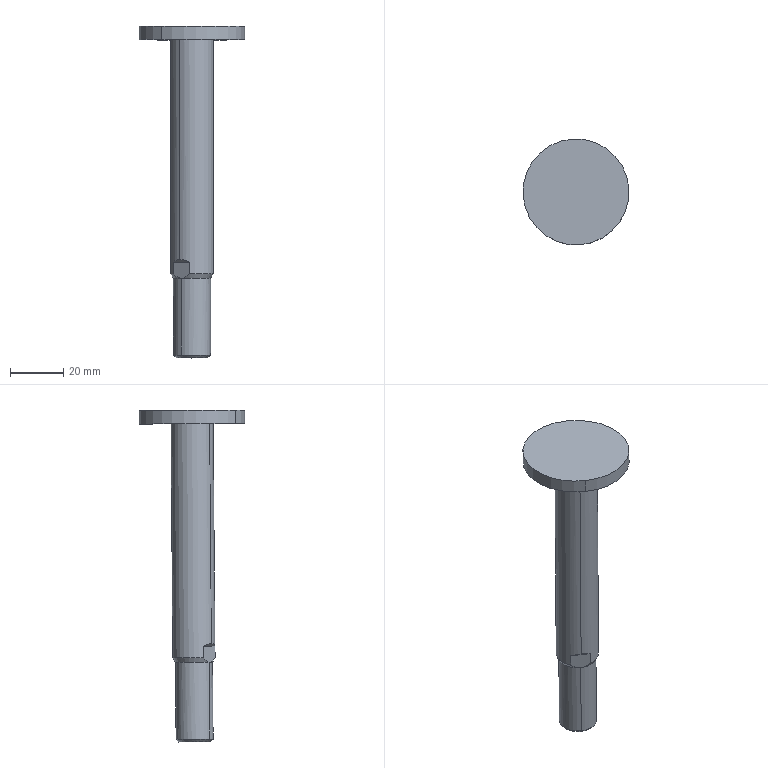Component | SolidWorks | CG1UN40-50Piston-1 | 1 solid | 17 faces | box 40 x 40.04 x 125.21 mm | volume 28878 mm3 | plane 7 | cylinder 6 | cone 4 | commonest cylinder face diameters 16 x2 40 x2 14 x2
STEP:
#1=CARTESIAN_POINT('',(8.156,4.289,0.9635));
#2=VERTEX_POINT('',#1);
#3=CARTESIAN_POINT('',(8.053,4.409,1.002));
#4=VERTEX_POINT('',#3);
#5=CARTESIAN_POINT('',(8.156,4.289,0.9635));
#6=CARTESIAN_POINT('',(8.132,4.338,0.9891));
#7=CARTESIAN_POINT('',(8.097,4.378,1.002));
#8=CARTESIAN_POINT('',(8.053,4.409,1.002));
#9=(BOUNDED_CURVE()B_SPLINE_CURVE(3,(#5,#6,#7,#8),.UNSPECIFIED.,.F.,.F.)B_SPLINE_CURVE_WITH_KNOTS((4,4),(5.778,6.283),.UNSPECIFIED.)CURVE()GEOMETRIC_REPRESENTATION_ITEM()RATIONAL_B_SPLINE_CURVE((1.,0.9788,0.9788,1.))REPRESENTATION_ITEM(''));
#10=EDGE_CURVE('',#2,#4,#9,.T.);
#11=ORIENTED_EDGE('',*,*,#10,.T.);
#12=CARTESIAN_POINT('',(8.053,4.435,4.27));
#13=VERTEX_POINT('',#12);
#14=CARTESIAN_POINT('',(8.053,4.42,2.439));
#15=DIRECTION('',(-0.,0.008055,1.));
#16=VECTOR('',#15,39.37);
#17=LINE('',#14,#16);
#18=EDGE_CURVE('',#4,#13,#17,.T.);
#19=ORIENTED_EDGE('',*,*,#18,.T.);
#20=CARTESIAN_POINT('',(7.695,3.917,4.274));
#21=VERTEX_POINT('',#20);
#22=CARTESIAN_POINT('',(7.874,4.176,4.272));
#23=DIRECTION('',(0.,-0.008055,-1.));
#24=DIRECTION('',(-0.5679,-0.823,0.00663));
#25=AXIS2_PLACEMENT_3D('',#22,#23,#24);
#26=CIRCLE('',#25,0.315);
#27=EDGE_CURVE('',#13,#21,#26,.T.);
#28=ORIENTED_EDGE('',*,*,#27,.T.);
#29=CARTESIAN_POINT('',(7.695,3.89,1.006));
#30=VERTEX_POINT('',#29);
#31=CARTESIAN_POINT('',(7.695,3.902,2.443));
#32=DIRECTION('',(-0.,0.008055,1.));
#33=VECTOR('',#32,39.37);
#34=LINE('',#31,#33);
#35=EDGE_CURVE('',#30,#21,#34,.T.);
#36=ORIENTED_EDGE('',*,*,#35,.F.);
#37=CARTESIAN_POINT('',(7.843,3.836,0.9672));
#38=VERTEX_POINT('',#37);
#39=CARTESIAN_POINT('',(7.695,3.89,1.006));
#40=CARTESIAN_POINT('',(7.739,3.86,1.006));
#41=CARTESIAN_POINT('',(7.79,3.841,0.9931));
#42=CARTESIAN_POINT('',(7.843,3.836,0.9672));
#43=(BOUNDED_CURVE()B_SPLINE_CURVE(3,(#39,#40,#41,#42),.UNSPECIFIED.,.F.,.T.)B_SPLINE_CURVE_WITH_KNOTS((4,4),(0.,0.5054),.UNSPECIFIED.)CURVE()GEOMETRIC_REPRESENTATION_ITEM()RATIONAL_B_SPLINE_CURVE((1.,0.9788,0.9788,1.))REPRESENTATION_ITEM(''));
#44=EDGE_CURVE('',#30,#38,#43,.T.);
#45=ORIENTED_EDGE('',*,*,#44,.T.);
#46=CARTESIAN_POINT('',(7.843,3.834,0.7992));
#47=VERTEX_POINT('',#46);
#48=CARTESIAN_POINT('',(7.843,3.848,2.444));
#49=DIRECTION('',(0.,-0.008055,-1.));
#50=VECTOR('',#49,39.37);
#51=LINE('',#48,#50);
#52=EDGE_CURVE('',#38,#47,#51,.T.);
#53=ORIENTED_EDGE('',*,*,#52,.T.);
#54=CARTESIAN_POINT('',(8.156,4.288,0.7955));
#55=VERTEX_POINT('',#54);
#56=CARTESIAN_POINT('',(7.874,4.148,0.7966));
#57=DIRECTION('',(-0.,0.008055,1.));
#58=DIRECTION('',(-0.5679,-0.823,0.00663));
#59=AXIS2_PLACEMENT_3D('',#56,#57,#58);
#60=CIRCLE('',#59,0.315);
#61=EDGE_CURVE('',#47,#55,#60,.T.);
#62=ORIENTED_EDGE('',*,*,#61,.T.);
#63=CARTESIAN_POINT('',(8.156,4.301,2.44));
#64=DIRECTION('',(-0.,0.008055,1.));
#65=VECTOR('',#64,39.37);
#66=LINE('',#63,#65);
#67=EDGE_CURVE('',#55,#2,#66,.T.);
#68=ORIENTED_EDGE('',*,*,#67,.T.);
#69=EDGE_LOOP('',(#11,#19,#28,#36,#45,#53,#62,#68));
#70=FACE_OUTER_BOUND('',#69,.T.);
#71=CARTESIAN_POINT('',(7.874,4.161,2.441));
#72=DIRECTION('',(-0.,0.008055,1.));
#73=DIRECTION('',(-0.5679,-0.823,0.00663));
#74=AXIS2_PLACEMENT_3D('',#71,#72,#73);
#75=CYLINDRICAL_SURFACE('',#74,0.315);
#76=ADVANCED_FACE('',(#70),#75,.T.);
#77=CARTESIAN_POINT('',(8.321,4.824,4.266));
#78=VERTEX_POINT('',#77);
#79=CARTESIAN_POINT('',(7.427,3.528,4.277));
#80=VERTEX_POINT('',#79);
#81=CARTESIAN_POINT('',(7.874,4.176,4.272));
#82=DIRECTION('',(0.,-0.008055,-1.));
#83=DIRECTION('',(-0.5679,-0.823,0.00663));
#84=AXIS2_PLACEMENT_3D('',#81,#82,#83);
#85=CIRCLE('',#84,0.7874);
#86=EDGE_CURVE('',#78,#80,#85,.T.);
#87=ORIENTED_EDGE('',*,*,#86,.F.);
#88=CARTESIAN_POINT('',(8.321,4.825,4.463));
#89=VERTEX_POINT('',#88);
#90=CARTESIAN_POINT('',(8.321,4.825,4.365));
#91=DIRECTION('',(-0.,0.008055,1.));
#92=VECTOR('',#91,39.37);
#93=LINE('',#90,#92);
#94=EDGE_CURVE('',#78,#89,#93,.T.);
#95=ORIENTED_EDGE('',*,*,#94,.T.);
#96=CARTESIAN_POINT('',(7.427,3.529,4.474));
#97=VERTEX_POINT('',#96);
#98=CARTESIAN_POINT('',(7.874,4.177,4.468));
#99=DIRECTION('',(0.,-0.008055,-1.));
#100=DIRECTION('',(-0.5679,-0.823,0.00663));
#101=AXIS2_PLACEMENT_3D('',#98,#99,#100);
#102=CIRCLE('',#101,0.7874);
#103=EDGE_CURVE('',#89,#97,#102,.T.);
#104=ORIENTED_EDGE('',*,*,#103,.T.);
#105=CARTESIAN_POINT('',(7.427,3.528,4.375));
#106=DIRECTION('',(-0.,0.008055,1.));
#107=VECTOR('',#106,39.37);
#108=LINE('',#105,#107);
#109=EDGE_CURVE('',#80,#97,#108,.T.);
#110=ORIENTED_EDGE('',*,*,#109,.F.);
#111=EDGE_LOOP('',(#87,#95,#104,#110));
#112=FACE_OUTER_BOUND('',#111,.T.);
#113=CARTESIAN_POINT('',(7.874,4.177,4.37));
#114=DIRECTION('',(-0.,0.008055,1.));
#115=DIRECTION('',(-0.5679,-0.823,0.00663));
#116=AXIS2_PLACEMENT_3D('',#113,#114,#115);
#117=CYLINDRICAL_SURFACE('',#116,0.7874);
#118=ADVANCED_FACE('',(#112),#117,.T.);
#119=CARTESIAN_POINT('',(8.101,3.982,-0.412));
#120=VERTEX_POINT('',#119);
#121=CARTESIAN_POINT('',(8.031,4.365,-0.4151));
#122=VERTEX_POINT('',#121);
#123=CARTESIAN_POINT('',(7.874,4.138,-0.4132));
#124=DIRECTION('',(-0.,0.008055,1.));
#125=DIRECTION('',(-0.5679,-0.823,0.00663));
#126=AXIS2_PLACEMENT_3D('',#123,#124,#125);
#127=CIRCLE('',#126,0.2756);
#128=EDGE_CURVE('',#120,#122,#127,.T.);
#129=ORIENTED_EDGE('',*,*,#128,.T.);
#130=CARTESIAN_POINT('',(8.031,4.374,0.7266));
#131=VERTEX_POINT('',#130);
#132=CARTESIAN_POINT('',(8.031,4.369,0.09672));
#133=DIRECTION('',(-0.,0.008055,1.));
#134=VECTOR('',#133,39.37);
#135=LINE('',#132,#134);
#136=EDGE_CURVE('',#122,#131,#135,.T.);
#137=ORIENTED_EDGE('',*,*,#136,.T.);
#138=CARTESIAN_POINT('',(7.717,3.92,0.7303));
#139=VERTEX_POINT('',#138);
#140=CARTESIAN_POINT('',(7.874,4.147,0.7285));
#141=DIRECTION('',(-0.,0.008055,1.));
#142=DIRECTION('',(-0.5679,-0.823,0.00663));
#143=AXIS2_PLACEMENT_3D('',#140,#141,#142);
#144=CIRCLE('',#143,0.2756);
#145=EDGE_CURVE('',#139,#131,#144,.T.);
#146=ORIENTED_EDGE('',*,*,#145,.F.);
#147=CARTESIAN_POINT('',(7.717,3.911,-0.4114));
#148=VERTEX_POINT('',#147);
#149=CARTESIAN_POINT('',(7.717,3.915,0.1004));
#150=DIRECTION('',(-0.,0.008055,1.));
#151=VECTOR('',#150,39.37);
#152=LINE('',#149,#151);
#153=EDGE_CURVE('',#148,#139,#152,.T.);
#154=ORIENTED_EDGE('',*,*,#153,.F.);
#155=CARTESIAN_POINT('',(7.874,4.138,-0.4132));
#156=DIRECTION('',(-0.,0.008055,1.));
#157=DIRECTION('',(-0.5679,-0.823,0.00663));
#158=AXIS2_PLACEMENT_3D('',#155,#156,#157);
#159=CIRCLE('',#158,0.2756);
#160=EDGE_CURVE('',#148,#120,#159,.T.);
#161=ORIENTED_EDGE('',*,*,#160,.T.);
#162=EDGE_LOOP('',(#129,#137,#146,#154,#161));
#163=FACE_OUTER_BOUND('',#162,.T.);
#164=CARTESIAN_POINT('',(7.874,4.142,0.09855));
#165=DIRECTION('',(-0.,0.008055,1.));
#166=DIRECTION('',(-0.5679,-0.823,0.00663));
#167=AXIS2_PLACEMENT_3D('',#164,#165,#166);
#168=CYLINDRICAL_SURFACE('',#167,0.2756);
#169=ADVANCED_FACE('',(#163),#168,.T.);
#170=CARTESIAN_POINT('',(8.068,4.004,-0.4515));
#171=VERTEX_POINT('',#170);
#172=CARTESIAN_POINT('',(7.68,4.272,-0.4537));
#173=VERTEX_POINT('',#172);
#174=CARTESIAN_POINT('',(7.874,4.138,-0.4526));
#175=DIRECTION('',(-0.,0.008055,1.));
#176=DIRECTION('',(0.8231,-0.5679,0.004575));
#177=AXIS2_PLACEMENT_3D('',#174,#175,#176);
#178=CIRCLE('',#177,0.2362);
#179=EDGE_CURVE('',#171,#173,#178,.T.);
#180=ORIENTED_EDGE('',*,*,#179,.T.);
#181=CARTESIAN_POINT('',(7.647,4.295,-0.4145));
#182=VERTEX_POINT('',#181);
#183=CARTESIAN_POINT('',(7.647,4.295,-0.4145));
#184=DIRECTION('',(-0.582,0.4073,0.7038));
#185=VECTOR('',#184,39.37);
#186=LINE('',#183,#185);
#187=EDGE_CURVE('',#173,#182,#186,.T.);
#188=ORIENTED_EDGE('',*,*,#187,.T.);
#189=CARTESIAN_POINT('',(7.874,4.138,-0.4132));
#190=DIRECTION('',(-0.,0.008055,1.));
#191=DIRECTION('',(-0.5679,-0.823,0.00663));
#192=AXIS2_PLACEMENT_3D('',#189,#190,#191);
#193=CIRCLE('',#192,0.2756);
#194=EDGE_CURVE('',#122,#182,#193,.T.);
#195=ORIENTED_EDGE('',*,*,#194,.F.);
#196=ORIENTED_EDGE('',*,*,#128,.F.);
#197=CARTESIAN_POINT('',(8.101,3.982,-0.412));
#198=DIRECTION('',(0.582,-0.3959,0.7103));
#199=VECTOR('',#198,39.37);
#200=LINE('',#197,#199);
#201=EDGE_CURVE('',#171,#120,#200,.T.);
#202=ORIENTED_EDGE('',*,*,#201,.F.);
#203=EDGE_LOOP('',(#180,#188,#195,#196,#202));
#204=FACE_OUTER_BOUND('',#203,.T.);
#205=CARTESIAN_POINT('',(7.874,4.138,-0.4132));
#206=DIRECTION('',(-0.,0.008055,1.));
#207=DIRECTION('',(0.8231,-0.5679,0.004575));
#208=AXIS2_PLACEMENT_3D('',#205,#206,#207);
#209=CONICAL_SURFACE('',#208,0.2756,0.7854);
#210=ADVANCED_FACE('',(#204),#209,.T.);
#211=ORIENTED_EDGE('',*,*,#18,.F.);
#212=CARTESIAN_POINT('',(7.905,4.463,0.9621));
#213=VERTEX_POINT('',#212);
#214=CARTESIAN_POINT('',(8.053,4.409,1.002));
#215=CARTESIAN_POINT('',(8.009,4.439,1.002));
#216=CARTESIAN_POINT('',(7.958,4.457,0.9881));
#217=CARTESIAN_POINT('',(7.905,4.463,0.9621));
#218=(BOUNDED_CURVE()B_SPLINE_CURVE(3,(#214,#215,#216,#217),.UNSPECIFIED.,.F.,.F.)B_SPLINE_CURVE_WITH_KNOTS((4,4),(-0.,0.5054),.UNSPECIFIED.)CURVE()GEOMETRIC_REPRESENTATION_ITEM()RATIONAL_B_SPLINE_CURVE((1.,0.9788,0.9788,1.))REPRESENTATION_ITEM(''));
#219=EDGE_CURVE('',#4,#213,#218,.T.);
#220=ORIENTED_EDGE('',*,*,#219,.T.);
#221=CARTESIAN_POINT('',(7.905,4.461,0.7941));
#222=VERTEX_POINT('',#221);
#223=CARTESIAN_POINT('',(7.905,4.474,2.438));
#224=DIRECTION('',(0.,-0.008055,-1.));
#225=VECTOR('',#224,39.37);
#226=LINE('',#223,#225);
#227=EDGE_CURVE('',#213,#222,#226,.T.);
#228=ORIENTED_EDGE('',*,*,#227,.T.);
#229=CARTESIAN_POINT('',(7.592,4.008,0.7978));
#230=VERTEX_POINT('',#229);
#231=CARTESIAN_POINT('',(7.874,4.148,0.7966));
#232=DIRECTION('',(-0.,0.008055,1.));
#233=DIRECTION('',(-0.5679,-0.823,0.00663));
#234=AXIS2_PLACEMENT_3D('',#231,#232,#233);
#235=CIRCLE('',#234,0.315);
#236=EDGE_CURVE('',#222,#230,#235,.T.);
#237=ORIENTED_EDGE('',*,*,#236,.T.);
#238=CARTESIAN_POINT('',(7.592,4.009,0.9658));
#239=VERTEX_POINT('',#238);
#240=CARTESIAN_POINT('',(7.592,4.021,2.442));
#241=DIRECTION('',(-0.,0.008055,1.));
#242=VECTOR('',#241,39.37);
#243=LINE('',#240,#242);
#244=EDGE_CURVE('',#230,#239,#243,.T.);
#245=ORIENTED_EDGE('',*,*,#244,.T.);
#246=CARTESIAN_POINT('',(7.592,4.009,0.9658));
#247=CARTESIAN_POINT('',(7.616,3.961,0.9921));
#248=CARTESIAN_POINT('',(7.651,3.921,1.006));
#249=CARTESIAN_POINT('',(7.695,3.89,1.006));
#250=(BOUNDED_CURVE()B_SPLINE_CURVE(3,(#246,#247,#248,#249),.UNSPECIFIED.,.F.,.T.)B_SPLINE_CURVE_WITH_KNOTS((4,4),(5.778,6.283),.UNSPECIFIED.)CURVE()GEOMETRIC_REPRESENTATION_ITEM()RATIONAL_B_SPLINE_CURVE((1.,0.9788,0.9788,1.))REPRESENTATION_ITEM(''));
#251=EDGE_CURVE('',#239,#30,#250,.T.);
#252=ORIENTED_EDGE('',*,*,#251,.T.);
#253=ORIENTED_EDGE('',*,*,#35,.T.);
#254=CARTESIAN_POINT('',(7.874,4.176,4.272));
#255=DIRECTION('',(0.,-0.008055,-1.));
#256=DIRECTION('',(-0.5679,-0.823,0.00663));
#257=AXIS2_PLACEMENT_3D('',#254,#255,#256);
#258=CIRCLE('',#257,0.315);
#259=EDGE_CURVE('',#21,#13,#258,.T.);
#260=ORIENTED_EDGE('',*,*,#259,.T.);
#261=EDGE_LOOP('',(#211,#220,#228,#237,#245,#252,#253,#260));
#262=FACE_OUTER_BOUND('',#261,.T.);
#263=CARTESIAN_POINT('',(7.874,4.161,2.441));
#264=DIRECTION('',(-0.,0.008055,1.));
#265=DIRECTION('',(-0.5679,-0.823,0.00663));
#266=AXIS2_PLACEMENT_3D('',#263,#264,#265);
#267=CYLINDRICAL_SURFACE('',#266,0.315);
#268=ADVANCED_FACE('',(#262),#267,.T.);
#269=CARTESIAN_POINT('',(7.874,4.176,4.272));
#270=DIRECTION('',(0.,-0.008055,-1.));
#271=DIRECTION('',(-0.5679,-0.823,0.00663));
#272=AXIS2_PLACEMENT_3D('',#269,#270,#271);
#273=CIRCLE('',#272,0.7874);
#274=EDGE_CURVE('',#80,#78,#273,.T.);
#275=ORIENTED_EDGE('',*,*,#274,.T.);
#276=ORIENTED_EDGE('',*,*,#86,.T.);
#277=EDGE_LOOP('',(#275,#276));
#278=FACE_OUTER_BOUND('',#277,.T.);
#279=ORIENTED_EDGE('',*,*,#259,.F.);
#280=ORIENTED_EDGE('',*,*,#27,.F.);
#281=EDGE_LOOP('',(#279,#280));
#282=FACE_BOUND('',#281,.T.);
#283=CARTESIAN_POINT('',(8.328,3.863,4.274));
#284=DIRECTION('',(0.,-0.008055,-1.));
#285=DIRECTION('',(0.5679,0.823,-0.00663));
#286=AXIS2_PLACEMENT_3D('',#283,#284,#285);
#287=PLANE('',#286);
#288=ADVANCED_FACE('',(#278,#282),#287,.T.);
#289=CARTESIAN_POINT('',(7.717,3.92,0.7303));
#290=CARTESIAN_POINT('',(7.706,3.929,0.7302));
#291=CARTESIAN_POINT('',(7.694,3.937,0.7321));
#292=CARTESIAN_POINT('',(7.672,3.952,0.7392));
#293=CARTESIAN_POINT('',(7.66,3.96,0.7444));
#294=CARTESIAN_POINT('',(7.64,3.974,0.7568));
#295=CARTESIAN_POINT('',(7.63,3.981,0.7641));
#296=CARTESIAN_POINT('',(7.61,3.995,0.78));
#297=CARTESIAN_POINT('',(7.601,4.001,0.7887));
#298=CARTESIAN_POINT('',(7.592,4.008,0.7978));
#299=B_SPLINE_CURVE_WITH_KNOTS('',3,(#289,#290,#291,#292,#293,#294,#295,#296,#297,#298),.UNSPECIFIED.,.F.,.F.,(4,2,2,2,4),(0.,0.001077,0.002154,0.003231,0.004308),.UNSPECIFIED.);
#300=EDGE_CURVE('',#139,#230,#299,.T.);
#301=ORIENTED_EDGE('',*,*,#300,.T.);
#302=ORIENTED_EDGE('',*,*,#236,.F.);
#303=CARTESIAN_POINT('',(7.905,4.461,0.7941));
#304=CARTESIAN_POINT('',(7.923,4.449,0.7759));
#305=CARTESIAN_POINT('',(7.942,4.435,0.7595));
#306=CARTESIAN_POINT('',(7.973,4.414,0.7408));
#307=CARTESIAN_POINT('',(7.984,4.406,0.7355));
#308=CARTESIAN_POINT('',(8.007,4.39,0.7285));
#309=CARTESIAN_POINT('',(8.019,4.382,0.7266));
#310=CARTESIAN_POINT('',(8.031,4.374,0.7266));
#311=B_SPLINE_CURVE_WITH_KNOTS('',3,(#303,#304,#305,#306,#307,#308,#309,#310),.UNSPECIFIED.,.F.,.F.,(4,2,2,4),(0.,0.002152,0.003229,0.004305),.UNSPECIFIED.);
#312=EDGE_CURVE('',#222,#131,#311,.T.);
#313=ORIENTED_EDGE('',*,*,#312,.T.);
#314=CARTESIAN_POINT('',(7.874,4.147,0.7285));
#315=DIRECTION('',(-0.,0.008055,1.));
#316=DIRECTION('',(-0.5679,-0.823,0.00663));
#317=AXIS2_PLACEMENT_3D('',#314,#315,#316);
#318=CIRCLE('',#317,0.2756);
#319=EDGE_CURVE('',#131,#139,#318,.T.);
#320=ORIENTED_EDGE('',*,*,#319,.T.);
#321=EDGE_LOOP('',(#301,#302,#313,#320));
#322=FACE_OUTER_BOUND('',#321,.T.);
#323=CARTESIAN_POINT('',(7.874,4.148,0.7966));
#324=DIRECTION('',(-0.,0.008055,1.));
#325=DIRECTION('',(-0.5679,-0.823,0.00663));
#326=AXIS2_PLACEMENT_3D('',#323,#324,#325);
#327=CONICAL_SURFACE('',#326,0.315,0.5236);
#328=ADVANCED_FACE('',(#322),#327,.T.);
#329=CARTESIAN_POINT('',(8.031,4.374,0.7266));
#330=CARTESIAN_POINT('',(8.042,4.366,0.7267));
#331=CARTESIAN_POINT('',(8.054,4.358,0.7287));
#332=CARTESIAN_POINT('',(8.076,4.342,0.736));
#333=CARTESIAN_POINT('',(8.088,4.335,0.7413));
#334=CARTESIAN_POINT('',(8.109,4.32,0.754));
#335=CARTESIAN_POINT('',(8.118,4.314,0.7614));
#336=CARTESIAN_POINT('',(8.138,4.3,0.7775));
#337=CARTESIAN_POINT('',(8.147,4.294,0.7863));
#338=CARTESIAN_POINT('',(8.156,4.288,0.7955));
#339=B_SPLINE_CURVE_WITH_KNOTS('',3,(#329,#330,#331,#332,#333,#334,#335,#336,#337,#338),.UNSPECIFIED.,.F.,.F.,(4,2,2,2,4),(0.,0.001077,0.002154,0.003231,0.004308),.UNSPECIFIED.);
#340=EDGE_CURVE('',#131,#55,#339,.T.);
#341=ORIENTED_EDGE('',*,*,#340,.F.);
#342=ORIENTED_EDGE('',*,*,#312,.F.);
#343=ORIENTED_EDGE('',*,*,#227,.F.);
#344=CARTESIAN_POINT('',(9.003,3.705,0.9682));
#345=DIRECTION('',(-0.8231,0.5679,-0.004575));
#346=VECTOR('',#345,39.37);
#347=LINE('',#344,#346);
#348=EDGE_CURVE('',#2,#213,#347,.T.);
#349=ORIENTED_EDGE('',*,*,#348,.F.);
#350=ORIENTED_EDGE('',*,*,#67,.F.);
#351=EDGE_LOOP('',(#341,#342,#343,#349,#350));
#352=FACE_OUTER_BOUND('',#351,.T.);
#353=CARTESIAN_POINT('',(9.003,3.705,0.9682));
#354=DIRECTION('',(-0.5679,-0.823,0.00663));
#355=DIRECTION('',(0.,-0.008055,-1.));
#356=AXIS2_PLACEMENT_3D('',#353,#354,#355);
#357=PLANE('',#356);
#358=ADVANCED_FACE('',(#352),#357,.F.);
#359=ORIENTED_EDGE('',*,*,#348,.T.);
#360=ORIENTED_EDGE('',*,*,#219,.F.);
#361=ORIENTED_EDGE('',*,*,#10,.F.);
#362=EDGE_LOOP('',(#359,#360,#361));
#363=FACE_OUTER_BOUND('',#362,.T.);
#364=CARTESIAN_POINT('',(9.114,3.869,1.164));
#365=DIRECTION('',(-0.4016,-0.5763,0.7118));
#366=DIRECTION('',(-0.4016,-0.5877,-0.7024));
#367=AXIS2_PLACEMENT_3D('',#364,#365,#366);
#368=PLANE('',#367);
#369=ADVANCED_FACE('',(#363),#368,.F.);
#370=CARTESIAN_POINT('',(7.843,3.834,0.7992));
#371=CARTESIAN_POINT('',(7.825,3.847,0.7807));
#372=CARTESIAN_POINT('',(7.806,3.86,0.7641));
#373=CARTESIAN_POINT('',(7.775,3.881,0.7451));
#374=CARTESIAN_POINT('',(7.764,3.889,0.7397));
#375=CARTESIAN_POINT('',(7.741,3.904,0.7324));
#376=CARTESIAN_POINT('',(7.729,3.912,0.7303));
#377=CARTESIAN_POINT('',(7.717,3.92,0.7303));
#378=B_SPLINE_CURVE_WITH_KNOTS('',3,(#370,#371,#372,#373,#374,#375,#376,#377),.UNSPECIFIED.,.F.,.F.,(4,2,2,4),(0.,0.002152,0.003229,0.004305),.UNSPECIFIED.);
#379=EDGE_CURVE('',#47,#139,#378,.T.);
#380=ORIENTED_EDGE('',*,*,#379,.T.);
#381=ORIENTED_EDGE('',*,*,#145,.T.);
#382=ORIENTED_EDGE('',*,*,#340,.T.);
#383=ORIENTED_EDGE('',*,*,#61,.F.);
#384=EDGE_LOOP('',(#380,#381,#382,#383));
#385=FACE_OUTER_BOUND('',#384,.T.);
#386=CARTESIAN_POINT('',(7.874,4.148,0.7966));
#387=DIRECTION('',(-0.,0.008055,1.));
#388=DIRECTION('',(-0.5679,-0.823,0.00663));
#389=AXIS2_PLACEMENT_3D('',#386,#387,#388);
#390=CONICAL_SURFACE('',#389,0.315,0.5236);
#391=ADVANCED_FACE('',(#385),#390,.T.);
#392=ORIENTED_EDGE('',*,*,#94,.F.);
#393=ORIENTED_EDGE('',*,*,#274,.F.);
#394=ORIENTED_EDGE('',*,*,#109,.T.);
#395=CARTESIAN_POINT('',(7.874,4.177,4.468));
#396=DIRECTION('',(0.,-0.008055,-1.));
#397=DIRECTION('',(-0.5679,-0.823,0.00663));
#398=AXIS2_PLACEMENT_3D('',#395,#396,#397);
#399=CIRCLE('',#398,0.7874);
#400=EDGE_CURVE('',#97,#89,#399,.T.);
#401=ORIENTED_EDGE('',*,*,#400,.T.);
#402=EDGE_LOOP('',(#392,#393,#394,#401));
#403=FACE_OUTER_BOUND('',#402,.T.);
#404=CARTESIAN_POINT('',(7.874,4.177,4.37));
#405=DIRECTION('',(-0.,0.008055,1.));
#406=DIRECTION('',(-0.5679,-0.823,0.00663));
#407=AXIS2_PLACEMENT_3D('',#404,#405,#406);
#408=CYLINDRICAL_SURFACE('',#407,0.7874);
#409=ADVANCED_FACE('',(#403),#408,.T.);
#410=ORIENTED_EDGE('',*,*,#300,.F.);
#411=ORIENTED_EDGE('',*,*,#379,.F.);
#412=ORIENTED_EDGE('',*,*,#52,.F.);
#413=CARTESIAN_POINT('',(8.69,3.252,0.9719));
#414=DIRECTION('',(0.8231,-0.5679,0.004575));
#415=VECTOR('',#414,39.37);
#416=LINE('',#413,#415);
#417=EDGE_CURVE('',#239,#38,#416,.T.);
#418=ORIENTED_EDGE('',*,*,#417,.F.);
#419=ORIENTED_EDGE('',*,*,#244,.F.);
#420=EDGE_LOOP('',(#410,#411,#412,#418,#419));
#421=FACE_OUTER_BOUND('',#420,.T.);
#422=CARTESIAN_POINT('',(8.69,3.24,-0.4454));
#423=DIRECTION('',(0.5679,0.823,-0.00663));
#424=DIRECTION('',(-0.,0.008055,1.));
#425=AXIS2_PLACEMENT_3D('',#422,#423,#424);
#426=PLANE('',#425);
#427=ADVANCED_FACE('',(#421),#426,.F.);
#428=ORIENTED_EDGE('',*,*,#417,.T.);
#429=ORIENTED_EDGE('',*,*,#44,.F.);
#430=ORIENTED_EDGE('',*,*,#251,.F.);
#431=EDGE_LOOP('',(#428,#429,#430));
#432=FACE_OUTER_BOUND('',#431,.T.);
#433=CARTESIAN_POINT('',(8.69,3.252,0.9719));
#434=DIRECTION('',(0.4016,0.5877,0.7024));
#435=DIRECTION('',(-0.4016,-0.5763,0.7118));
#436=AXIS2_PLACEMENT_3D('',#433,#434,#435);
#437=PLANE('',#436);
#438=ADVANCED_FACE('',(#432),#437,.F.);
#439=ORIENTED_EDGE('',*,*,#136,.F.);
#440=ORIENTED_EDGE('',*,*,#194,.T.);
#441=CARTESIAN_POINT('',(7.874,4.138,-0.4132));
#442=DIRECTION('',(-0.,0.008055,1.));
#443=DIRECTION('',(-0.5679,-0.823,0.00663));
#444=AXIS2_PLACEMENT_3D('',#441,#442,#443);
#445=CIRCLE('',#444,0.2756);
#446=EDGE_CURVE('',#182,#148,#445,.T.);
#447=ORIENTED_EDGE('',*,*,#446,.T.);
#448=ORIENTED_EDGE('',*,*,#153,.T.);
#449=ORIENTED_EDGE('',*,*,#319,.F.);
#450=EDGE_LOOP('',(#439,#440,#447,#448,#449));
#451=FACE_OUTER_BOUND('',#450,.T.);
#452=CARTESIAN_POINT('',(7.874,4.142,0.09855));
#453=DIRECTION('',(-0.,0.008055,1.));
#454=DIRECTION('',(-0.5679,-0.823,0.00663));
#455=AXIS2_PLACEMENT_3D('',#452,#453,#454);
#456=CYLINDRICAL_SURFACE('',#455,0.2756);
#457=ADVANCED_FACE('',(#451),#456,.T.);
#458=ORIENTED_EDGE('',*,*,#400,.F.);
#459=ORIENTED_EDGE('',*,*,#103,.F.);
#460=EDGE_LOOP('',(#458,#459));
#461=FACE_OUTER_BOUND('',#460,.T.);
#462=CARTESIAN_POINT('',(8.198,3.954,4.47));
#463=DIRECTION('',(-0.,0.008055,1.));
#464=DIRECTION('',(-0.5679,-0.823,0.00663));
#465=AXIS2_PLACEMENT_3D('',#462,#463,#464);
#466=PLANE('',#465);
#467=ADVANCED_FACE('',(#461),#466,.T.);
#468=ORIENTED_EDGE('',*,*,#187,.F.);
#469=CARTESIAN_POINT('',(7.874,4.138,-0.4526));
#470=DIRECTION('',(-0.,0.008055,1.));
#471=DIRECTION('',(0.8231,-0.5679,0.004575));
#472=AXIS2_PLACEMENT_3D('',#469,#470,#471);
#473=CIRCLE('',#472,0.2362);
#474=EDGE_CURVE('',#173,#171,#473,.T.);
#475=ORIENTED_EDGE('',*,*,#474,.T.);
#476=ORIENTED_EDGE('',*,*,#201,.T.);
#477=ORIENTED_EDGE('',*,*,#160,.F.);
#478=ORIENTED_EDGE('',*,*,#446,.F.);
#479=EDGE_LOOP('',(#468,#475,#476,#477,#478));
#480=FACE_OUTER_BOUND('',#479,.T.);
#481=CARTESIAN_POINT('',(7.874,4.138,-0.4132));
#482=DIRECTION('',(-0.,0.008055,1.));
#483=DIRECTION('',(0.8231,-0.5679,0.004575));
#484=AXIS2_PLACEMENT_3D('',#481,#482,#483);
#485=CONICAL_SURFACE('',#484,0.2756,0.7854);
#486=ADVANCED_FACE('',(#480),#485,.T.);
#487=ORIENTED_EDGE('',*,*,#179,.F.);
#488=ORIENTED_EDGE('',*,*,#474,.F.);
#489=EDGE_LOOP('',(#487,#488));
#490=FACE_OUTER_BOUND('',#489,.T.);
#491=CARTESIAN_POINT('',(7.807,4.041,-0.4518));
#492=DIRECTION('',(0.,-0.008055,-1.));
#493=DIRECTION('',(0.5679,0.823,-0.00663));
#494=AXIS2_PLACEMENT_3D('',#491,#492,#493);
#495=PLANE('',#494);
#496=ADVANCED_FACE('',(#490),#495,.T.);
#497=CLOSED_SHELL('',(#76,#118,#169,#210,#268,#288,#328,#358,#369,#391,#409,#427,#438,#457,#467,#486,#496));
#498=MANIFOLD_SOLID_BREP('',#497);
#499=CARTESIAN_POINT('',(0.,0.,0.));
#500=DIRECTION('',(0.,0.,1.));
#501=DIRECTION('',(1.,0.,0.));
#502=AXIS2_PLACEMENT_3D('',#499,#500,#501);
#503=(LENGTH_UNIT()NAMED_UNIT(*)SI_UNIT($,.METRE.));
#504=LENGTH_MEASURE_WITH_UNIT(LENGTH_MEASURE(0.0254),#503);
#505=DIMENSIONAL_EXPONENTS(1.,0.,0.,0.,0.,0.,0.);
#506=(CONVERSION_BASED_UNIT('',#504)LENGTH_UNIT()NAMED_UNIT(#505));
#507=UNCERTAINTY_MEASURE_WITH_UNIT(LENGTH_MEASURE(0.00001),#506,'','');
#508=(NAMED_UNIT(*)PLANE_ANGLE_UNIT()SI_UNIT($,.RADIAN.));
#509=(NAMED_UNIT(*)SI_UNIT($,.STERADIAN.)SOLID_ANGLE_UNIT());
#510=(GEOMETRIC_REPRESENTATION_CONTEXT(3)GLOBAL_UNCERTAINTY_ASSIGNED_CONTEXT((#507))GLOBAL_UNIT_ASSIGNED_CONTEXT((#506,#508,#509))REPRESENTATION_CONTEXT('',''));
#511=ADVANCED_BREP_SHAPE_REPRESENTATION('',(#498,#502),#510);
#512=COLOUR_RGB('',0.7922,0.8196,0.9333);
#513=FILL_AREA_STYLE_COLOUR('',#512);
#514=FILL_AREA_STYLE('',(#513));
#515=SURFACE_STYLE_FILL_AREA(#514);
#516=SURFACE_SIDE_STYLE('',(#515));
#517=SURFACE_STYLE_USAGE(.BOTH.,#516);
#518=PRESENTATION_STYLE_ASSIGNMENT((#517));
#519=STYLED_ITEM('',(#518),#498);
#520=(LENGTH_UNIT()NAMED_UNIT(*)SI_UNIT($,.METRE.));
#521=LENGTH_MEASURE_WITH_UNIT(LENGTH_MEASURE(0.0254),#520);
#522=DIMENSIONAL_EXPONENTS(1.,0.,0.,0.,0.,0.,0.);
#523=(CONVERSION_BASED_UNIT('',#521)LENGTH_UNIT()NAMED_UNIT(#522));
#524=UNCERTAINTY_MEASURE_WITH_UNIT(LENGTH_MEASURE(0.00001),#523,'','');
#525=(NAMED_UNIT(*)PLANE_ANGLE_UNIT()SI_UNIT($,.RADIAN.));
#526=(NAMED_UNIT(*)SI_UNIT($,.STERADIAN.)SOLID_ANGLE_UNIT());
#527=(GEOMETRIC_REPRESENTATION_CONTEXT(3)GLOBAL_UNCERTAINTY_ASSIGNED_CONTEXT((#524))GLOBAL_UNIT_ASSIGNED_CONTEXT((#523,#525,#526))REPRESENTATION_CONTEXT('',''));
#528=MECHANICAL_DESIGN_GEOMETRIC_PRESENTATION_REPRESENTATION('',(#519),#527);
#529=PRESENTATION_LAYER_ASSIGNMENT('','',(#519));